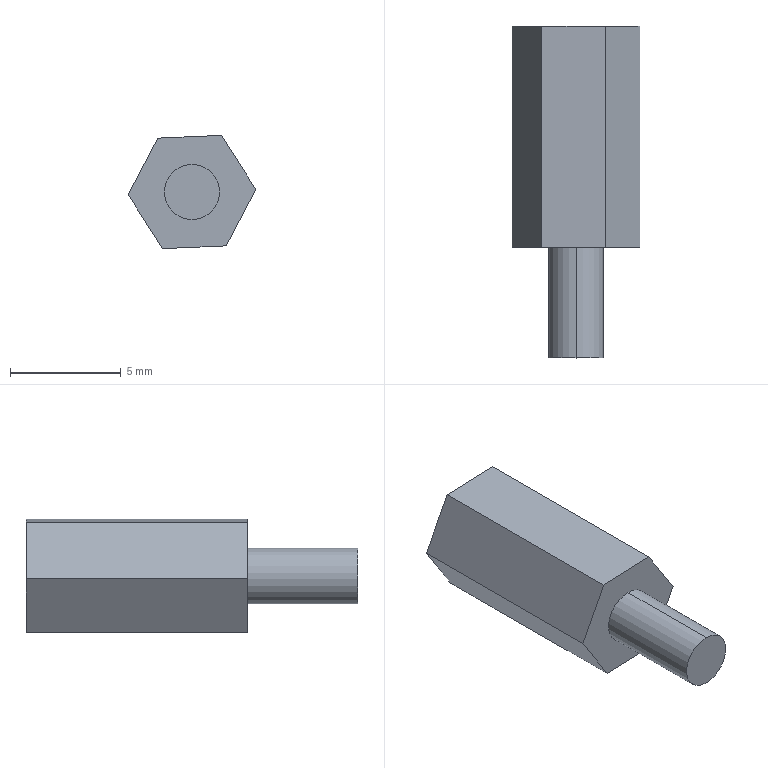Component | SolidWorks | Screw-2 | 1 solid | 14 faces | box 5.77 x 15 x 5.12 mm | volume 217 mm3 | plane 10 | cylinder 4 | commonest cylinder face diameters 2.5 x4
build123d program:
from build123d import *

# Parameters (mm, degrees)
BOSS_EXTRUDE2_DEPTH = 10
SKETCH2_R           = 1.25
BOSS_EXTRUDE3_DEPTH = 5
SKETCH3_R           = 1.25
CUT_EXTRUDE1_DEPTH  = 5


with BuildPart() as part:
    # Sketch1 → Boss-Extrude2 (new body)
    with BuildSketch(Plane(origin=(0, 0, 0), x_dir=(1, 0, 0), z_dir=(0, 1, 0))):
        Polygon((2.884, 0.1259), (1.333, 2.561), (-1.551, 2.435), (-2.884, -0.1259), (-1.333, -2.561), (1.551, -2.435), align=None)
    extrude(amount=BOSS_EXTRUDE2_DEPTH)

    # Sketch2 → Boss-Extrude3 (add)
    with BuildSketch(Plane(origin=(0, 10, 0), x_dir=(1, 0, 0), z_dir=(0, 1, 0))):
        with Locations(Location((0, 0, 0), (0, 0, 270))):
            Circle(SKETCH2_R)
    extrude(amount=BOSS_EXTRUDE3_DEPTH)

    # Sketch3 → Cut-Extrude1 (cut)
    with BuildSketch(Plane.XZ):
        with Locations(Location((0, 0, 0), (0, 0, 90))):
            Circle(SKETCH3_R)
    extrude(amount=-CUT_EXTRUDE1_DEPTH, mode=Mode.SUBTRACT)


solid = part.part

# Placed as in the assembly
solid = solid.moved(Location((-24.045, 16.631, 48), (180, 0, 0)))
STEP:
#1=COLOUR_RGB('',0.7922,0.8196,0.9333);
#2=FILL_AREA_STYLE_COLOUR('',#1);
#3=FILL_AREA_STYLE('',(#2));
#4=SURFACE_STYLE_FILL_AREA(#3);
#5=SURFACE_SIDE_STYLE('',(#4));
#6=SURFACE_STYLE_USAGE(.BOTH.,#5);
#7=PRESENTATION_STYLE_ASSIGNMENT((#6));
#8=CARTESIAN_POINT('',(-0.9467,0.4579,1.939));
#9=VERTEX_POINT('',#8);
#10=CARTESIAN_POINT('',(-0.9467,0.4579,1.841));
#11=VERTEX_POINT('',#10);
#12=CARTESIAN_POINT('',(-0.9467,0.4579,1.89));
#13=DIRECTION('',(-0.,1.,0.));
#14=DIRECTION('',(0.,0.,-1.));
#15=AXIS2_PLACEMENT_3D('',#12,#13,#14);
#16=CIRCLE('',#15,0.04921);
#17=EDGE_CURVE('',#9,#11,#16,.T.);
#18=ORIENTED_EDGE('',*,*,#17,.F.);
#19=CARTESIAN_POINT('',(-0.9467,0.6548,1.939));
#20=VERTEX_POINT('',#19);
#21=CARTESIAN_POINT('',(-0.9467,0.4579,1.939));
#22=DIRECTION('',(-0.,1.,0.));
#23=VECTOR('',#22,39.37);
#24=LINE('',#21,#23);
#25=EDGE_CURVE('',#9,#20,#24,.T.);
#26=ORIENTED_EDGE('',*,*,#25,.T.);
#27=CARTESIAN_POINT('',(-0.9467,0.6548,1.841));
#28=VERTEX_POINT('',#27);
#29=CARTESIAN_POINT('',(-0.9467,0.6548,1.89));
#30=DIRECTION('',(-0.,1.,0.));
#31=DIRECTION('',(0.,0.,-1.));
#32=AXIS2_PLACEMENT_3D('',#29,#30,#31);
#33=CIRCLE('',#32,0.04921);
#34=EDGE_CURVE('',#20,#28,#33,.T.);
#35=ORIENTED_EDGE('',*,*,#34,.T.);
#36=CARTESIAN_POINT('',(-0.9467,0.4579,1.841));
#37=DIRECTION('',(-0.,1.,0.));
#38=VECTOR('',#37,39.37);
#39=LINE('',#36,#38);
#40=EDGE_CURVE('',#11,#28,#39,.T.);
#41=ORIENTED_EDGE('',*,*,#40,.F.);
#42=EDGE_LOOP('',(#18,#26,#35,#41));
#43=FACE_OUTER_BOUND('',#42,.T.);
#44=CARTESIAN_POINT('',(-0.9467,0.4579,1.89));
#45=DIRECTION('',(-0.,1.,0.));
#46=DIRECTION('',(0.,0.,-1.));
#47=AXIS2_PLACEMENT_3D('',#44,#45,#46);
#48=CYLINDRICAL_SURFACE('',#47,0.04921);
#49=ADVANCED_FACE('',(#43),#48,.F.);
#50=CARTESIAN_POINT('',(-0.9467,0.06421,1.939));
#51=VERTEX_POINT('',#50);
#52=CARTESIAN_POINT('',(-0.9467,0.06421,1.841));
#53=VERTEX_POINT('',#52);
#54=CARTESIAN_POINT('',(-0.9467,0.06421,1.89));
#55=DIRECTION('',(0.,-1.,0.));
#56=DIRECTION('',(0.,0.,1.));
#57=AXIS2_PLACEMENT_3D('',#54,#55,#56);
#58=CIRCLE('',#57,0.04921);
#59=EDGE_CURVE('',#51,#53,#58,.T.);
#60=ORIENTED_EDGE('',*,*,#59,.F.);
#61=CARTESIAN_POINT('',(-0.9467,0.2611,1.939));
#62=VERTEX_POINT('',#61);
#63=CARTESIAN_POINT('',(-0.9467,0.06421,1.939));
#64=DIRECTION('',(-0.,1.,0.));
#65=VECTOR('',#64,39.37);
#66=LINE('',#63,#65);
#67=EDGE_CURVE('',#51,#62,#66,.T.);
#68=ORIENTED_EDGE('',*,*,#67,.T.);
#69=CARTESIAN_POINT('',(-0.9467,0.2611,1.841));
#70=VERTEX_POINT('',#69);
#71=CARTESIAN_POINT('',(-0.9467,0.2611,1.89));
#72=DIRECTION('',(0.,-1.,0.));
#73=DIRECTION('',(0.,0.,1.));
#74=AXIS2_PLACEMENT_3D('',#71,#72,#73);
#75=CIRCLE('',#74,0.04921);
#76=EDGE_CURVE('',#62,#70,#75,.T.);
#77=ORIENTED_EDGE('',*,*,#76,.T.);
#78=CARTESIAN_POINT('',(-0.9467,0.06421,1.841));
#79=DIRECTION('',(-0.,1.,0.));
#80=VECTOR('',#79,39.37);
#81=LINE('',#78,#80);
#82=EDGE_CURVE('',#53,#70,#81,.T.);
#83=ORIENTED_EDGE('',*,*,#82,.F.);
#84=EDGE_LOOP('',(#60,#68,#77,#83));
#85=FACE_OUTER_BOUND('',#84,.T.);
#86=CARTESIAN_POINT('',(-0.9467,0.06421,1.89));
#87=DIRECTION('',(-0.,1.,0.));
#88=DIRECTION('',(0.,0.,-1.));
#89=AXIS2_PLACEMENT_3D('',#86,#87,#88);
#90=CYLINDRICAL_SURFACE('',#89,0.04921);
#91=ADVANCED_FACE('',(#85),#90,.T.);
#92=CARTESIAN_POINT('',(-1.008,0.2611,1.986));
#93=VERTEX_POINT('',#92);
#94=CARTESIAN_POINT('',(-1.06,0.2611,1.885));
#95=VERTEX_POINT('',#94);
#96=CARTESIAN_POINT('',(-1.008,0.2611,1.986));
#97=DIRECTION('',(-0.4617,-0.,-0.887));
#98=VECTOR('',#97,39.37);
#99=LINE('',#96,#98);
#100=EDGE_CURVE('',#93,#95,#99,.T.);
#101=ORIENTED_EDGE('',*,*,#100,.T.);
#102=CARTESIAN_POINT('',(-0.9991,0.2611,1.789));
#103=VERTEX_POINT('',#102);
#104=CARTESIAN_POINT('',(-1.06,0.2611,1.885));
#105=DIRECTION('',(0.5373,0.,-0.8434));
#106=VECTOR('',#105,39.37);
#107=LINE('',#104,#106);
#108=EDGE_CURVE('',#95,#103,#107,.T.);
#109=ORIENTED_EDGE('',*,*,#108,.T.);
#110=CARTESIAN_POINT('',(-0.8856,0.2611,1.794));
#111=VERTEX_POINT('',#110);
#112=CARTESIAN_POINT('',(-0.9991,0.2611,1.789));
#113=DIRECTION('',(0.999,0.,0.04362));
#114=VECTOR('',#113,39.37);
#115=LINE('',#112,#114);
#116=EDGE_CURVE('',#103,#111,#115,.T.);
#117=ORIENTED_EDGE('',*,*,#116,.T.);
#118=CARTESIAN_POINT('',(-0.8331,0.2611,1.895));
#119=VERTEX_POINT('',#118);
#120=CARTESIAN_POINT('',(-0.8856,0.2611,1.794));
#121=DIRECTION('',(0.4617,0.,0.887));
#122=VECTOR('',#121,39.37);
#123=LINE('',#120,#122);
#124=EDGE_CURVE('',#111,#119,#123,.T.);
#125=ORIENTED_EDGE('',*,*,#124,.T.);
#126=CARTESIAN_POINT('',(-0.8942,0.2611,1.991));
#127=VERTEX_POINT('',#126);
#128=CARTESIAN_POINT('',(-0.8331,0.2611,1.895));
#129=DIRECTION('',(-0.5373,-0.,0.8434));
#130=VECTOR('',#129,39.37);
#131=LINE('',#128,#130);
#132=EDGE_CURVE('',#119,#127,#131,.T.);
#133=ORIENTED_EDGE('',*,*,#132,.T.);
#134=CARTESIAN_POINT('',(-0.8942,0.2611,1.991));
#135=DIRECTION('',(-0.999,-0.,-0.04362));
#136=VECTOR('',#135,39.37);
#137=LINE('',#134,#136);
#138=EDGE_CURVE('',#127,#93,#137,.T.);
#139=ORIENTED_EDGE('',*,*,#138,.T.);
#140=EDGE_LOOP('',(#101,#109,#117,#125,#133,#139));
#141=FACE_OUTER_BOUND('',#140,.T.);
#142=CARTESIAN_POINT('',(-0.9467,0.2611,1.89));
#143=DIRECTION('',(0.,-1.,0.));
#144=DIRECTION('',(0.,0.,1.));
#145=AXIS2_PLACEMENT_3D('',#142,#143,#144);
#146=CIRCLE('',#145,0.04921);
#147=EDGE_CURVE('',#70,#62,#146,.T.);
#148=ORIENTED_EDGE('',*,*,#147,.F.);
#149=ORIENTED_EDGE('',*,*,#76,.F.);
#150=EDGE_LOOP('',(#148,#149));
#151=FACE_BOUND('',#150,.T.);
#152=CARTESIAN_POINT('',(-0.9467,0.2611,1.89));
#153=DIRECTION('',(0.,-1.,0.));
#154=DIRECTION('',(0.,0.,1.));
#155=AXIS2_PLACEMENT_3D('',#152,#153,#154);
#156=PLANE('',#155);
#157=ADVANCED_FACE('',(#141,#151),#156,.T.);
#158=CARTESIAN_POINT('',(-1.008,0.6548,1.986));
#159=VERTEX_POINT('',#158);
#160=CARTESIAN_POINT('',(-1.06,0.6548,1.885));
#161=VERTEX_POINT('',#160);
#162=CARTESIAN_POINT('',(-1.008,0.6548,1.986));
#163=DIRECTION('',(-0.4617,-0.,-0.887));
#164=VECTOR('',#163,39.37);
#165=LINE('',#162,#164);
#166=EDGE_CURVE('',#159,#161,#165,.T.);
#167=ORIENTED_EDGE('',*,*,#166,.T.);
#168=CARTESIAN_POINT('',(-1.06,0.2611,1.885));
#169=DIRECTION('',(-0.,1.,0.));
#170=VECTOR('',#169,39.37);
#171=LINE('',#168,#170);
#172=EDGE_CURVE('',#95,#161,#171,.T.);
#173=ORIENTED_EDGE('',*,*,#172,.F.);
#174=ORIENTED_EDGE('',*,*,#100,.F.);
#175=CARTESIAN_POINT('',(-1.008,0.2611,1.986));
#176=DIRECTION('',(-0.,1.,0.));
#177=VECTOR('',#176,39.37);
#178=LINE('',#175,#177);
#179=EDGE_CURVE('',#93,#159,#178,.T.);
#180=ORIENTED_EDGE('',*,*,#179,.T.);
#181=EDGE_LOOP('',(#167,#173,#174,#180));
#182=FACE_OUTER_BOUND('',#181,.T.);
#183=CARTESIAN_POINT('',(-1.008,0.2611,1.986));
#184=DIRECTION('',(0.887,0.,-0.4617));
#185=DIRECTION('',(0.4617,0.,0.887));
#186=AXIS2_PLACEMENT_3D('',#183,#184,#185);
#187=PLANE('',#186);
#188=ADVANCED_FACE('',(#182),#187,.F.);
#189=CARTESIAN_POINT('',(-0.9991,0.6548,1.789));
#190=VERTEX_POINT('',#189);
#191=CARTESIAN_POINT('',(-1.06,0.6548,1.885));
#192=DIRECTION('',(0.5373,0.,-0.8434));
#193=VECTOR('',#192,39.37);
#194=LINE('',#191,#193);
#195=EDGE_CURVE('',#161,#190,#194,.T.);
#196=ORIENTED_EDGE('',*,*,#195,.T.);
#197=CARTESIAN_POINT('',(-0.9991,0.2611,1.789));
#198=DIRECTION('',(-0.,1.,0.));
#199=VECTOR('',#198,39.37);
#200=LINE('',#197,#199);
#201=EDGE_CURVE('',#103,#190,#200,.T.);
#202=ORIENTED_EDGE('',*,*,#201,.F.);
#203=ORIENTED_EDGE('',*,*,#108,.F.);
#204=ORIENTED_EDGE('',*,*,#172,.T.);
#205=EDGE_LOOP('',(#196,#202,#203,#204));
#206=FACE_OUTER_BOUND('',#205,.T.);
#207=CARTESIAN_POINT('',(-1.06,0.2611,1.885));
#208=DIRECTION('',(0.8434,0.,0.5373));
#209=DIRECTION('',(-0.5373,-0.,0.8434));
#210=AXIS2_PLACEMENT_3D('',#207,#208,#209);
#211=PLANE('',#210);
#212=ADVANCED_FACE('',(#206),#211,.F.);
#213=CARTESIAN_POINT('',(-0.8856,0.6548,1.794));
#214=VERTEX_POINT('',#213);
#215=CARTESIAN_POINT('',(-0.9991,0.6548,1.789));
#216=DIRECTION('',(0.999,0.,0.04362));
#217=VECTOR('',#216,39.37);
#218=LINE('',#215,#217);
#219=EDGE_CURVE('',#190,#214,#218,.T.);
#220=ORIENTED_EDGE('',*,*,#219,.T.);
#221=CARTESIAN_POINT('',(-0.8856,0.2611,1.794));
#222=DIRECTION('',(-0.,1.,0.));
#223=VECTOR('',#222,39.37);
#224=LINE('',#221,#223);
#225=EDGE_CURVE('',#111,#214,#224,.T.);
#226=ORIENTED_EDGE('',*,*,#225,.F.);
#227=ORIENTED_EDGE('',*,*,#116,.F.);
#228=ORIENTED_EDGE('',*,*,#201,.T.);
#229=EDGE_LOOP('',(#220,#226,#227,#228));
#230=FACE_OUTER_BOUND('',#229,.T.);
#231=CARTESIAN_POINT('',(-0.9991,0.2611,1.789));
#232=DIRECTION('',(-0.04362,-0.,0.999));
#233=DIRECTION('',(-0.999,-0.,-0.04362));
#234=AXIS2_PLACEMENT_3D('',#231,#232,#233);
#235=PLANE('',#234);
#236=ADVANCED_FACE('',(#230),#235,.F.);
#237=CARTESIAN_POINT('',(-0.8331,0.6548,1.895));
#238=VERTEX_POINT('',#237);
#239=CARTESIAN_POINT('',(-0.8856,0.6548,1.794));
#240=DIRECTION('',(0.4617,0.,0.887));
#241=VECTOR('',#240,39.37);
#242=LINE('',#239,#241);
#243=EDGE_CURVE('',#214,#238,#242,.T.);
#244=ORIENTED_EDGE('',*,*,#243,.T.);
#245=CARTESIAN_POINT('',(-0.8331,0.2611,1.895));
#246=DIRECTION('',(-0.,1.,0.));
#247=VECTOR('',#246,39.37);
#248=LINE('',#245,#247);
#249=EDGE_CURVE('',#119,#238,#248,.T.);
#250=ORIENTED_EDGE('',*,*,#249,.F.);
#251=ORIENTED_EDGE('',*,*,#124,.F.);
#252=ORIENTED_EDGE('',*,*,#225,.T.);
#253=EDGE_LOOP('',(#244,#250,#251,#252));
#254=FACE_OUTER_BOUND('',#253,.T.);
#255=CARTESIAN_POINT('',(-0.8856,0.2611,1.794));
#256=DIRECTION('',(-0.887,-0.,0.4617));
#257=DIRECTION('',(-0.4617,-0.,-0.887));
#258=AXIS2_PLACEMENT_3D('',#255,#256,#257);
#259=PLANE('',#258);
#260=ADVANCED_FACE('',(#254),#259,.F.);
#261=CARTESIAN_POINT('',(-0.8942,0.6548,1.991));
#262=VERTEX_POINT('',#261);
#263=CARTESIAN_POINT('',(-0.8331,0.6548,1.895));
#264=DIRECTION('',(-0.5373,-0.,0.8434));
#265=VECTOR('',#264,39.37);
#266=LINE('',#263,#265);
#267=EDGE_CURVE('',#238,#262,#266,.T.);
#268=ORIENTED_EDGE('',*,*,#267,.T.);
#269=CARTESIAN_POINT('',(-0.8942,0.2611,1.991));
#270=DIRECTION('',(-0.,1.,0.));
#271=VECTOR('',#270,39.37);
#272=LINE('',#269,#271);
#273=EDGE_CURVE('',#127,#262,#272,.T.);
#274=ORIENTED_EDGE('',*,*,#273,.F.);
#275=ORIENTED_EDGE('',*,*,#132,.F.);
#276=ORIENTED_EDGE('',*,*,#249,.T.);
#277=EDGE_LOOP('',(#268,#274,#275,#276));
#278=FACE_OUTER_BOUND('',#277,.T.);
#279=CARTESIAN_POINT('',(-0.8331,0.2611,1.895));
#280=DIRECTION('',(-0.8434,-0.,-0.5373));
#281=DIRECTION('',(0.5373,0.,-0.8434));
#282=AXIS2_PLACEMENT_3D('',#279,#280,#281);
#283=PLANE('',#282);
#284=ADVANCED_FACE('',(#278),#283,.F.);
#285=CARTESIAN_POINT('',(-0.8942,0.6548,1.991));
#286=DIRECTION('',(-0.999,-0.,-0.04362));
#287=VECTOR('',#286,39.37);
#288=LINE('',#285,#287);
#289=EDGE_CURVE('',#262,#159,#288,.T.);
#290=ORIENTED_EDGE('',*,*,#289,.T.);
#291=ORIENTED_EDGE('',*,*,#179,.F.);
#292=ORIENTED_EDGE('',*,*,#138,.F.);
#293=ORIENTED_EDGE('',*,*,#273,.T.);
#294=EDGE_LOOP('',(#290,#291,#292,#293));
#295=FACE_OUTER_BOUND('',#294,.T.);
#296=CARTESIAN_POINT('',(-0.8942,0.2611,1.991));
#297=DIRECTION('',(0.04362,0.,-0.999));
#298=DIRECTION('',(0.999,0.,0.04362));
#299=AXIS2_PLACEMENT_3D('',#296,#297,#298);
#300=PLANE('',#299);
#301=ADVANCED_FACE('',(#295),#300,.F.);
#302=CARTESIAN_POINT('',(-0.9467,0.6548,1.89));
#303=DIRECTION('',(-0.,1.,0.));
#304=DIRECTION('',(0.,0.,-1.));
#305=AXIS2_PLACEMENT_3D('',#302,#303,#304);
#306=CIRCLE('',#305,0.04921);
#307=EDGE_CURVE('',#28,#20,#306,.T.);
#308=ORIENTED_EDGE('',*,*,#307,.F.);
#309=ORIENTED_EDGE('',*,*,#34,.F.);
#310=EDGE_LOOP('',(#308,#309));
#311=FACE_BOUND('',#310,.T.);
#312=ORIENTED_EDGE('',*,*,#166,.F.);
#313=ORIENTED_EDGE('',*,*,#289,.F.);
#314=ORIENTED_EDGE('',*,*,#267,.F.);
#315=ORIENTED_EDGE('',*,*,#243,.F.);
#316=ORIENTED_EDGE('',*,*,#219,.F.);
#317=ORIENTED_EDGE('',*,*,#195,.F.);
#318=EDGE_LOOP('',(#312,#313,#314,#315,#316,#317));
#319=FACE_OUTER_BOUND('',#318,.T.);
#320=CARTESIAN_POINT('',(-0.9467,0.6548,1.89));
#321=DIRECTION('',(0.,-1.,0.));
#322=DIRECTION('',(0.,0.,1.));
#323=AXIS2_PLACEMENT_3D('',#320,#321,#322);
#324=PLANE('',#323);
#325=ADVANCED_FACE('',(#311,#319),#324,.F.);
#326=ORIENTED_EDGE('',*,*,#67,.F.);
#327=CARTESIAN_POINT('',(-0.9467,0.06421,1.89));
#328=DIRECTION('',(0.,-1.,0.));
#329=DIRECTION('',(0.,0.,1.));
#330=AXIS2_PLACEMENT_3D('',#327,#328,#329);
#331=CIRCLE('',#330,0.04921);
#332=EDGE_CURVE('',#53,#51,#331,.T.);
#333=ORIENTED_EDGE('',*,*,#332,.F.);
#334=ORIENTED_EDGE('',*,*,#82,.T.);
#335=ORIENTED_EDGE('',*,*,#147,.T.);
#336=EDGE_LOOP('',(#326,#333,#334,#335));
#337=FACE_OUTER_BOUND('',#336,.T.);
#338=CARTESIAN_POINT('',(-0.9467,0.06421,1.89));
#339=DIRECTION('',(-0.,1.,0.));
#340=DIRECTION('',(0.,0.,-1.));
#341=AXIS2_PLACEMENT_3D('',#338,#339,#340);
#342=CYLINDRICAL_SURFACE('',#341,0.04921);
#343=ADVANCED_FACE('',(#337),#342,.T.);
#344=ORIENTED_EDGE('',*,*,#332,.T.);
#345=ORIENTED_EDGE('',*,*,#59,.T.);
#346=EDGE_LOOP('',(#344,#345));
#347=FACE_OUTER_BOUND('',#346,.T.);
#348=CARTESIAN_POINT('',(-0.9467,0.06421,1.89));
#349=DIRECTION('',(0.,-1.,0.));
#350=DIRECTION('',(0.,0.,1.));
#351=AXIS2_PLACEMENT_3D('',#348,#349,#350);
#352=PLANE('',#351);
#353=ADVANCED_FACE('',(#347),#352,.T.);
#354=ORIENTED_EDGE('',*,*,#25,.F.);
#355=CARTESIAN_POINT('',(-0.9467,0.4579,1.89));
#356=DIRECTION('',(-0.,1.,0.));
#357=DIRECTION('',(0.,0.,-1.));
#358=AXIS2_PLACEMENT_3D('',#355,#356,#357);
#359=CIRCLE('',#358,0.04921);
#360=EDGE_CURVE('',#11,#9,#359,.T.);
#361=ORIENTED_EDGE('',*,*,#360,.F.);
#362=ORIENTED_EDGE('',*,*,#40,.T.);
#363=ORIENTED_EDGE('',*,*,#307,.T.);
#364=EDGE_LOOP('',(#354,#361,#362,#363));
#365=FACE_OUTER_BOUND('',#364,.T.);
#366=CARTESIAN_POINT('',(-0.9467,0.4579,1.89));
#367=DIRECTION('',(-0.,1.,0.));
#368=DIRECTION('',(0.,0.,-1.));
#369=AXIS2_PLACEMENT_3D('',#366,#367,#368);
#370=CYLINDRICAL_SURFACE('',#369,0.04921);
#371=ADVANCED_FACE('',(#365),#370,.F.);
#372=ORIENTED_EDGE('',*,*,#360,.T.);
#373=ORIENTED_EDGE('',*,*,#17,.T.);
#374=EDGE_LOOP('',(#372,#373));
#375=FACE_OUTER_BOUND('',#374,.T.);
#376=CARTESIAN_POINT('',(-0.9467,0.4579,1.89));
#377=DIRECTION('',(-0.,1.,0.));
#378=DIRECTION('',(0.,0.,-1.));
#379=AXIS2_PLACEMENT_3D('',#376,#377,#378);
#380=PLANE('',#379);
#381=ADVANCED_FACE('',(#375),#380,.T.);
#382=CLOSED_SHELL('',(#49,#91,#157,#188,#212,#236,#260,#284,#301,#325,#343,#353,#371,#381));
#383=MANIFOLD_SOLID_BREP('',#382);
#384=STYLED_ITEM('',(#7),#383);
#385=PRESENTATION_LAYER_ASSIGNMENT('','',(#384));
#386=CARTESIAN_POINT('',(0.,0.,0.));
#387=DIRECTION('',(0.,0.,1.));
#388=DIRECTION('',(1.,0.,0.));
#389=AXIS2_PLACEMENT_3D('',#386,#387,#388);
#390=(LENGTH_UNIT()NAMED_UNIT(*)SI_UNIT($,.METRE.));
#391=LENGTH_MEASURE_WITH_UNIT(LENGTH_MEASURE(0.0254),#390);
#392=DIMENSIONAL_EXPONENTS(1.,0.,0.,0.,0.,0.,0.);
#393=(CONVERSION_BASED_UNIT('',#391)LENGTH_UNIT()NAMED_UNIT(#392));
#394=UNCERTAINTY_MEASURE_WITH_UNIT(LENGTH_MEASURE(0.00001),#393,'','');
#395=(NAMED_UNIT(*)PLANE_ANGLE_UNIT()SI_UNIT($,.RADIAN.));
#396=(NAMED_UNIT(*)SI_UNIT($,.STERADIAN.)SOLID_ANGLE_UNIT());
#397=(GEOMETRIC_REPRESENTATION_CONTEXT(3)GLOBAL_UNCERTAINTY_ASSIGNED_CONTEXT((#394))GLOBAL_UNIT_ASSIGNED_CONTEXT((#393,#395,#396))REPRESENTATION_CONTEXT('',''));
#398=ADVANCED_BREP_SHAPE_REPRESENTATION('',(#383,#389),#397);
#399=(LENGTH_UNIT()NAMED_UNIT(*)SI_UNIT($,.METRE.));
#400=LENGTH_MEASURE_WITH_UNIT(LENGTH_MEASURE(0.0254),#399);
#401=DIMENSIONAL_EXPONENTS(1.,0.,0.,0.,0.,0.,0.);
#402=(CONVERSION_BASED_UNIT('',#400)LENGTH_UNIT()NAMED_UNIT(#401));
#403=UNCERTAINTY_MEASURE_WITH_UNIT(LENGTH_MEASURE(0.00001),#402,'','');
#404=(NAMED_UNIT(*)PLANE_ANGLE_UNIT()SI_UNIT($,.RADIAN.));
#405=(NAMED_UNIT(*)SI_UNIT($,.STERADIAN.)SOLID_ANGLE_UNIT());
#406=(GEOMETRIC_REPRESENTATION_CONTEXT(3)GLOBAL_UNCERTAINTY_ASSIGNED_CONTEXT((#403))GLOBAL_UNIT_ASSIGNED_CONTEXT((#402,#404,#405))REPRESENTATION_CONTEXT('',''));
#407=MECHANICAL_DESIGN_GEOMETRIC_PRESENTATION_REPRESENTATION('',(#384),#406);